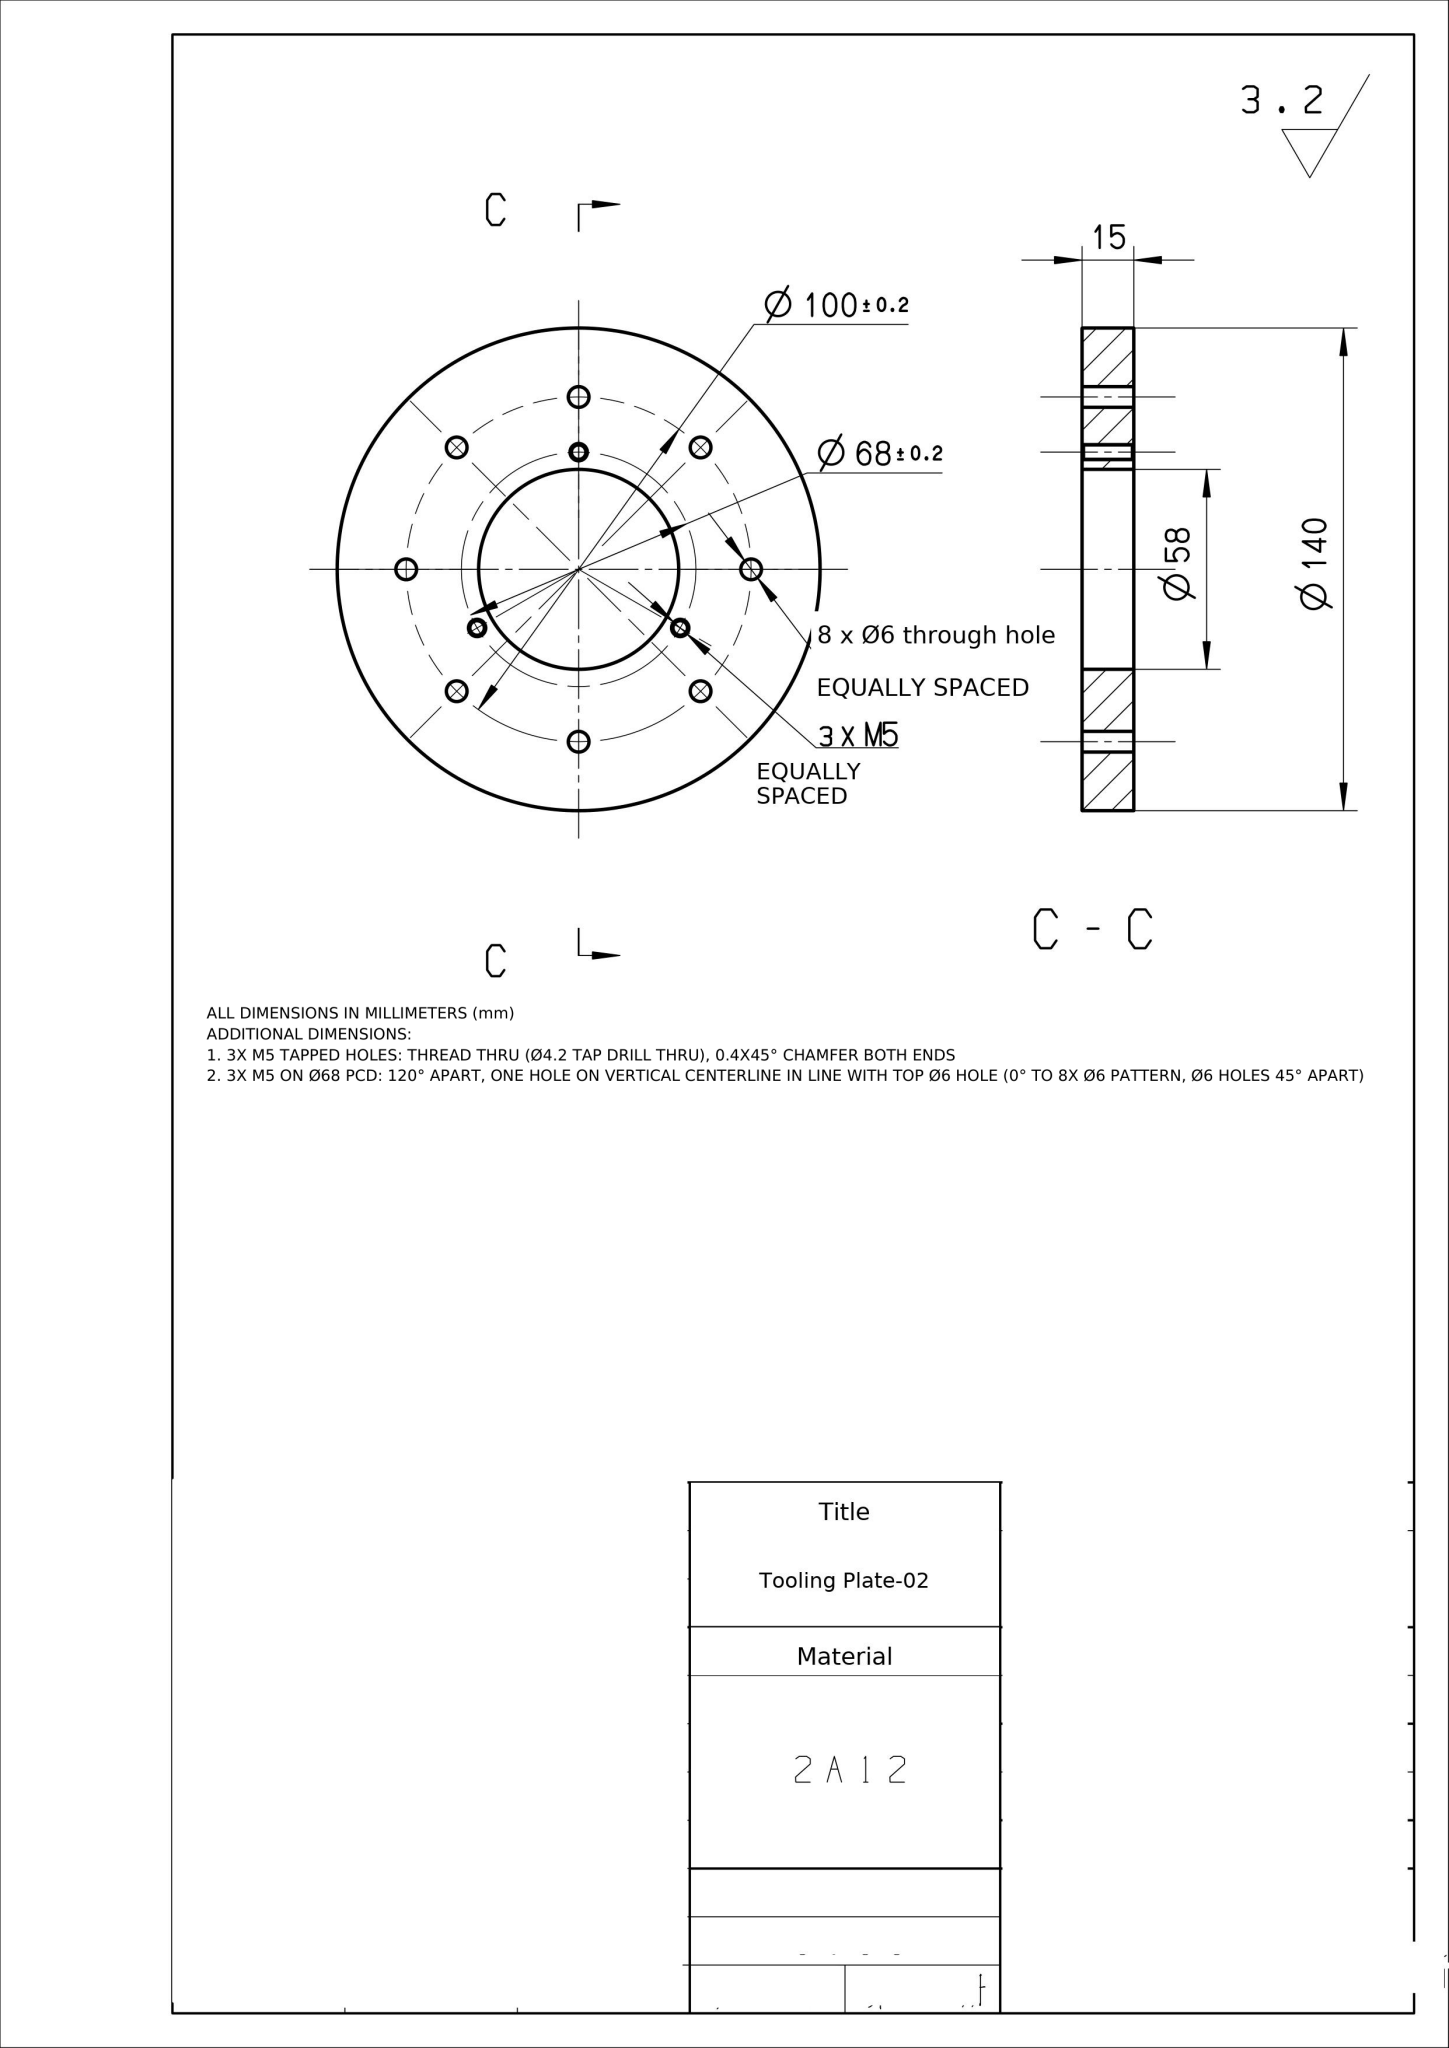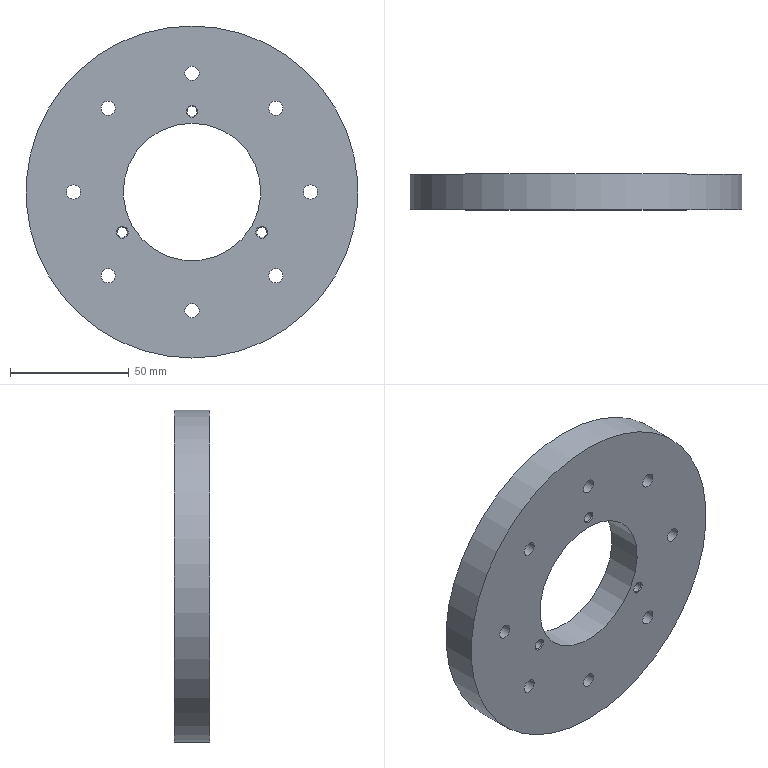Part | NX | mm | 1 solid | 21 faces | box 140 x 15 x 140 mm | volume 187253 mm3 | cylinder 13 | cone 6 | plane 2 | commonest cylinder face diameters 6 x8 4.2 x3 58 x1 140 x1